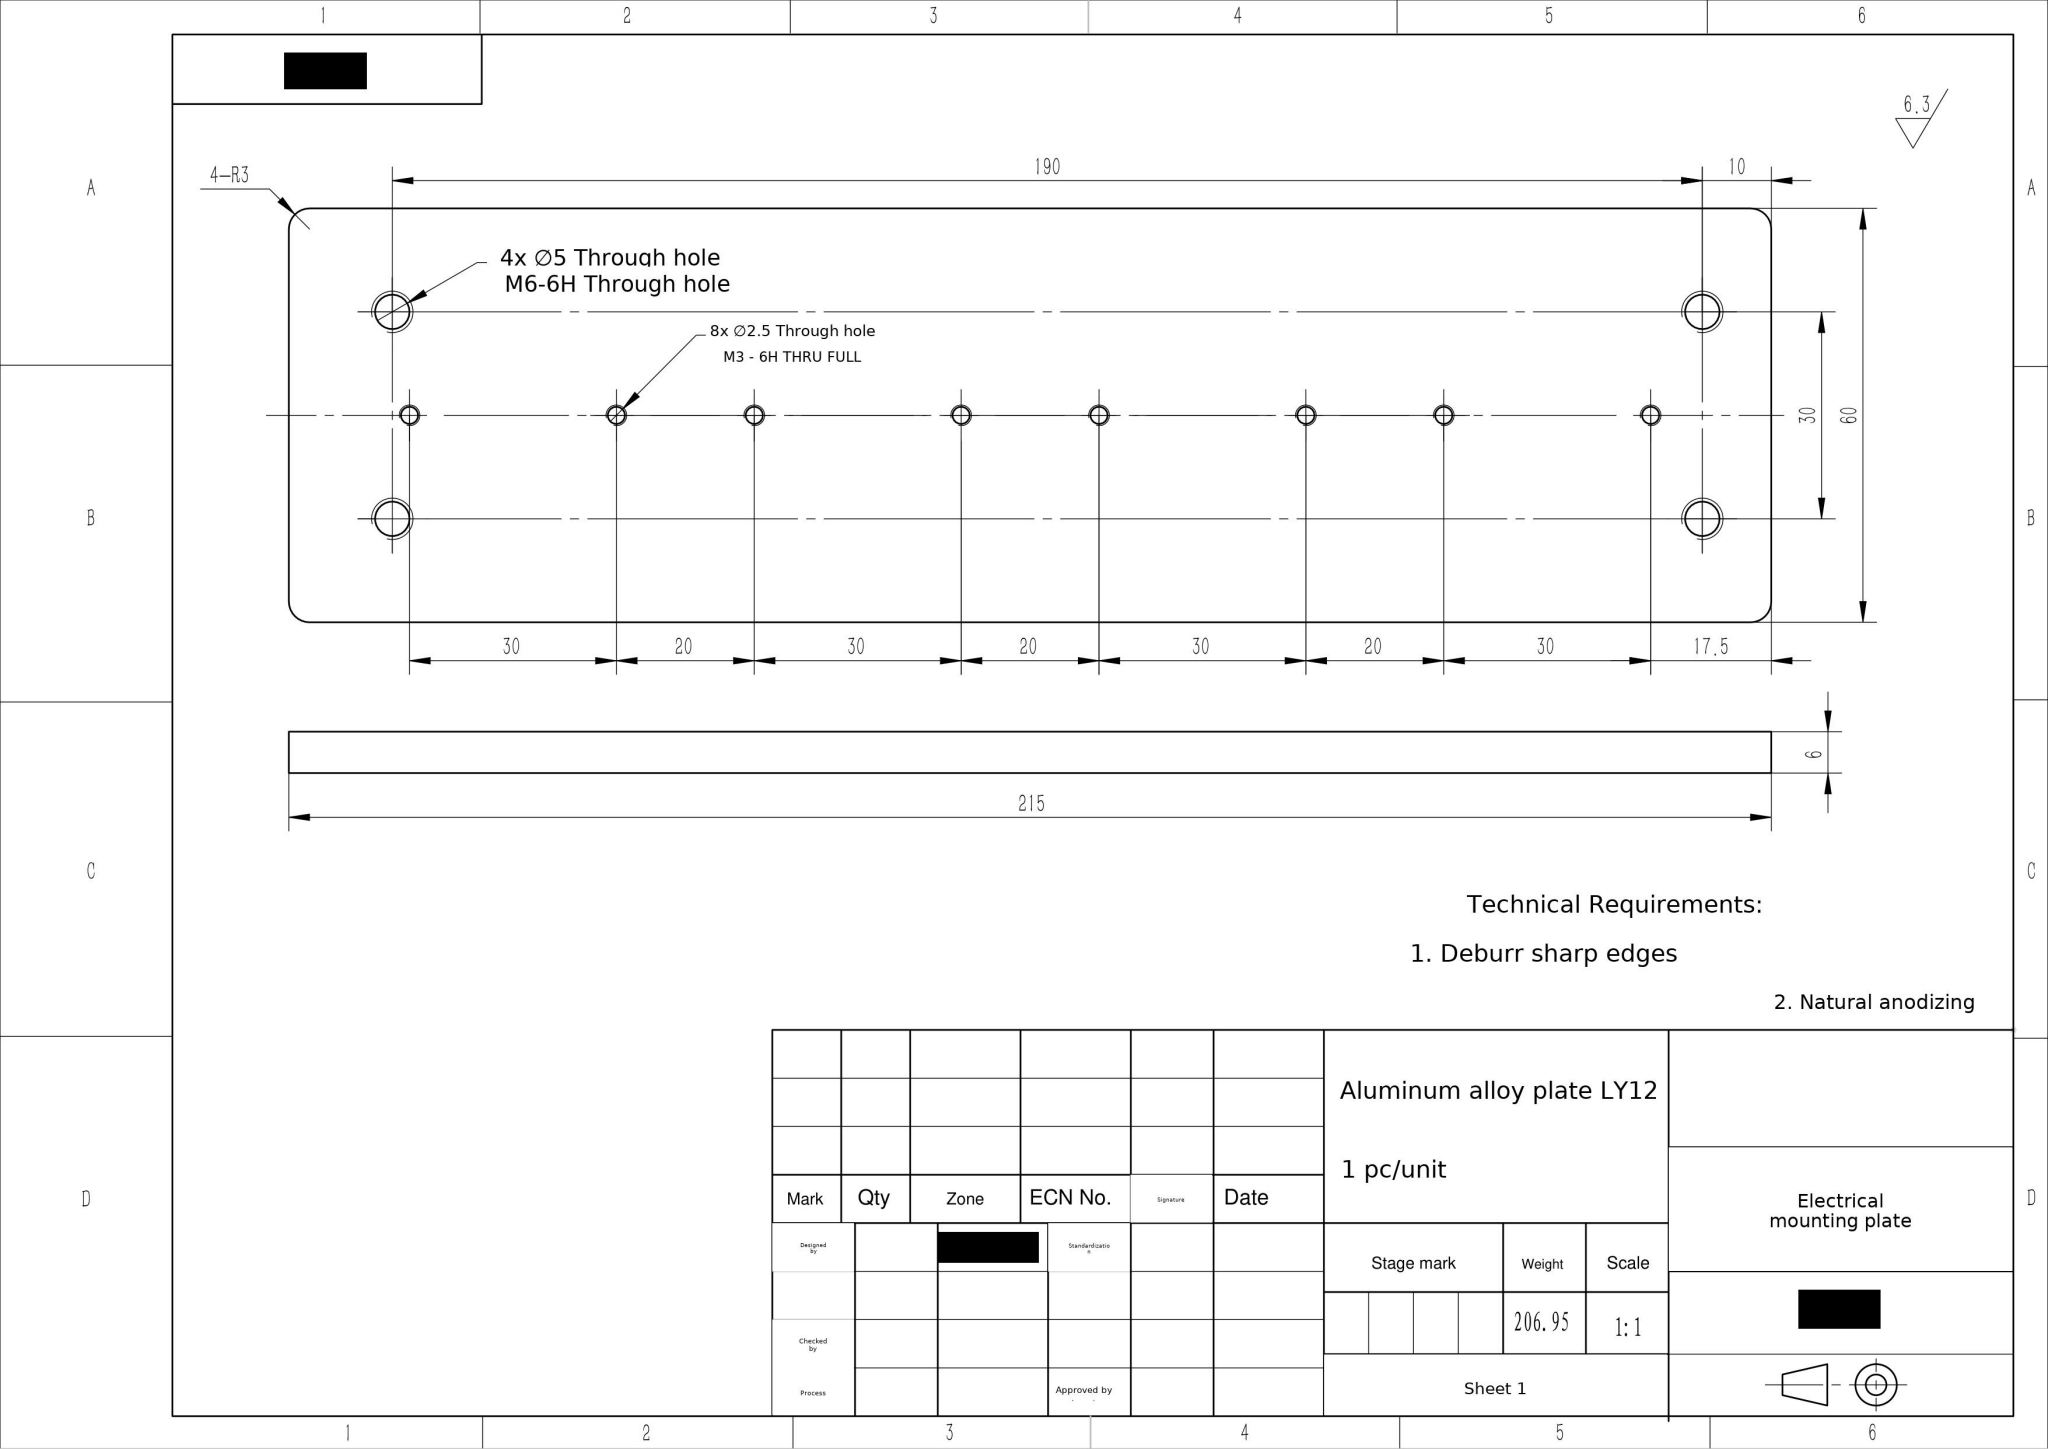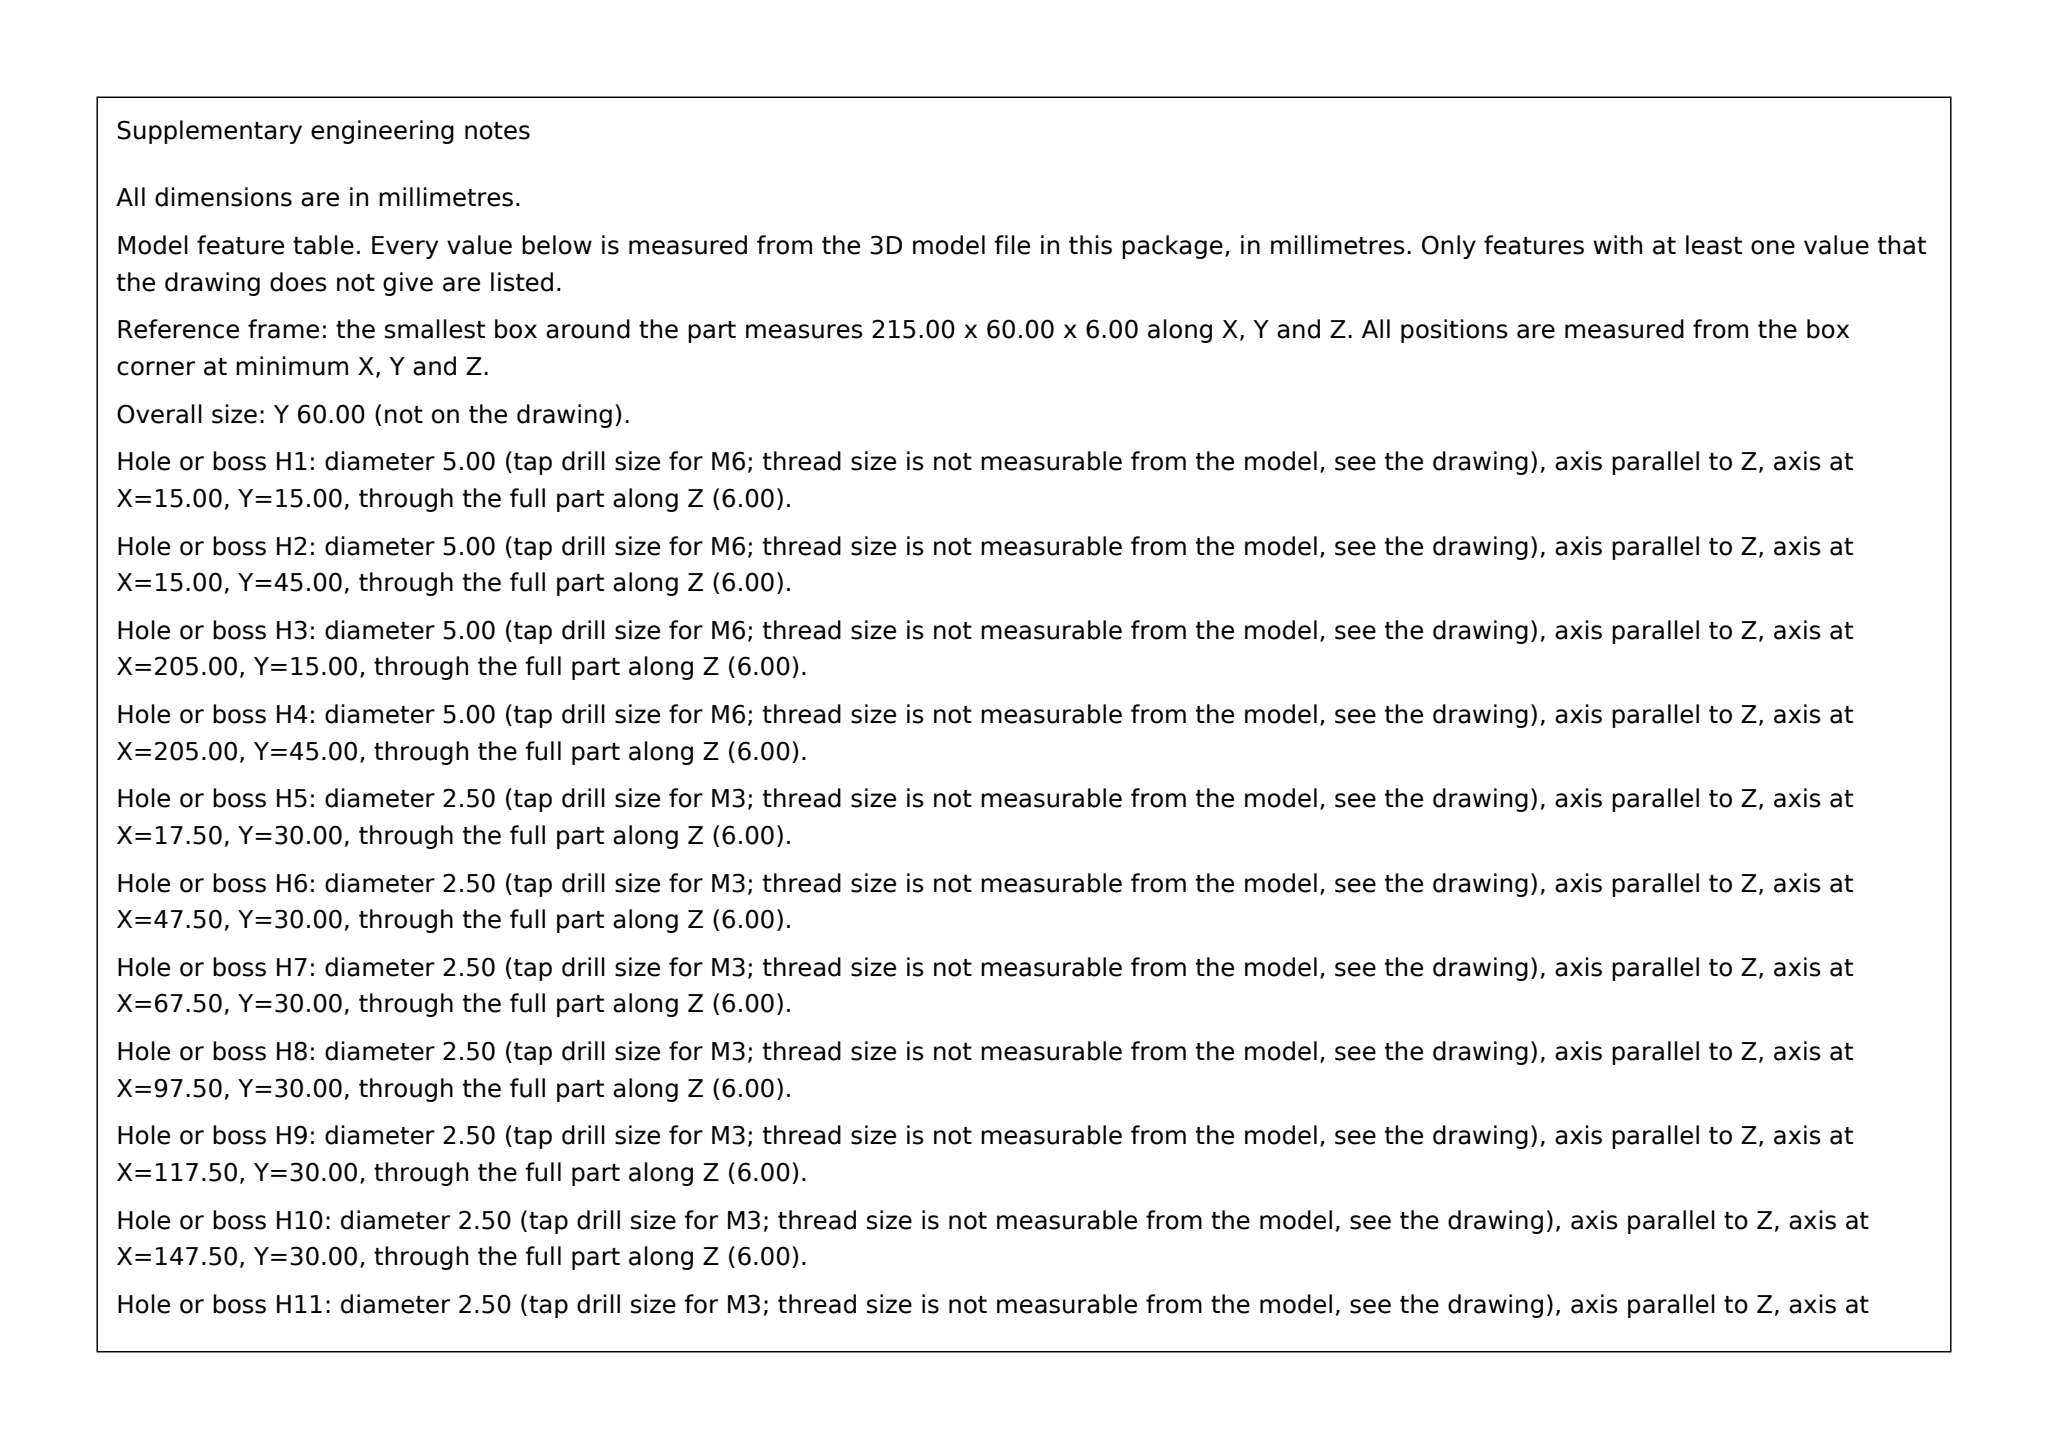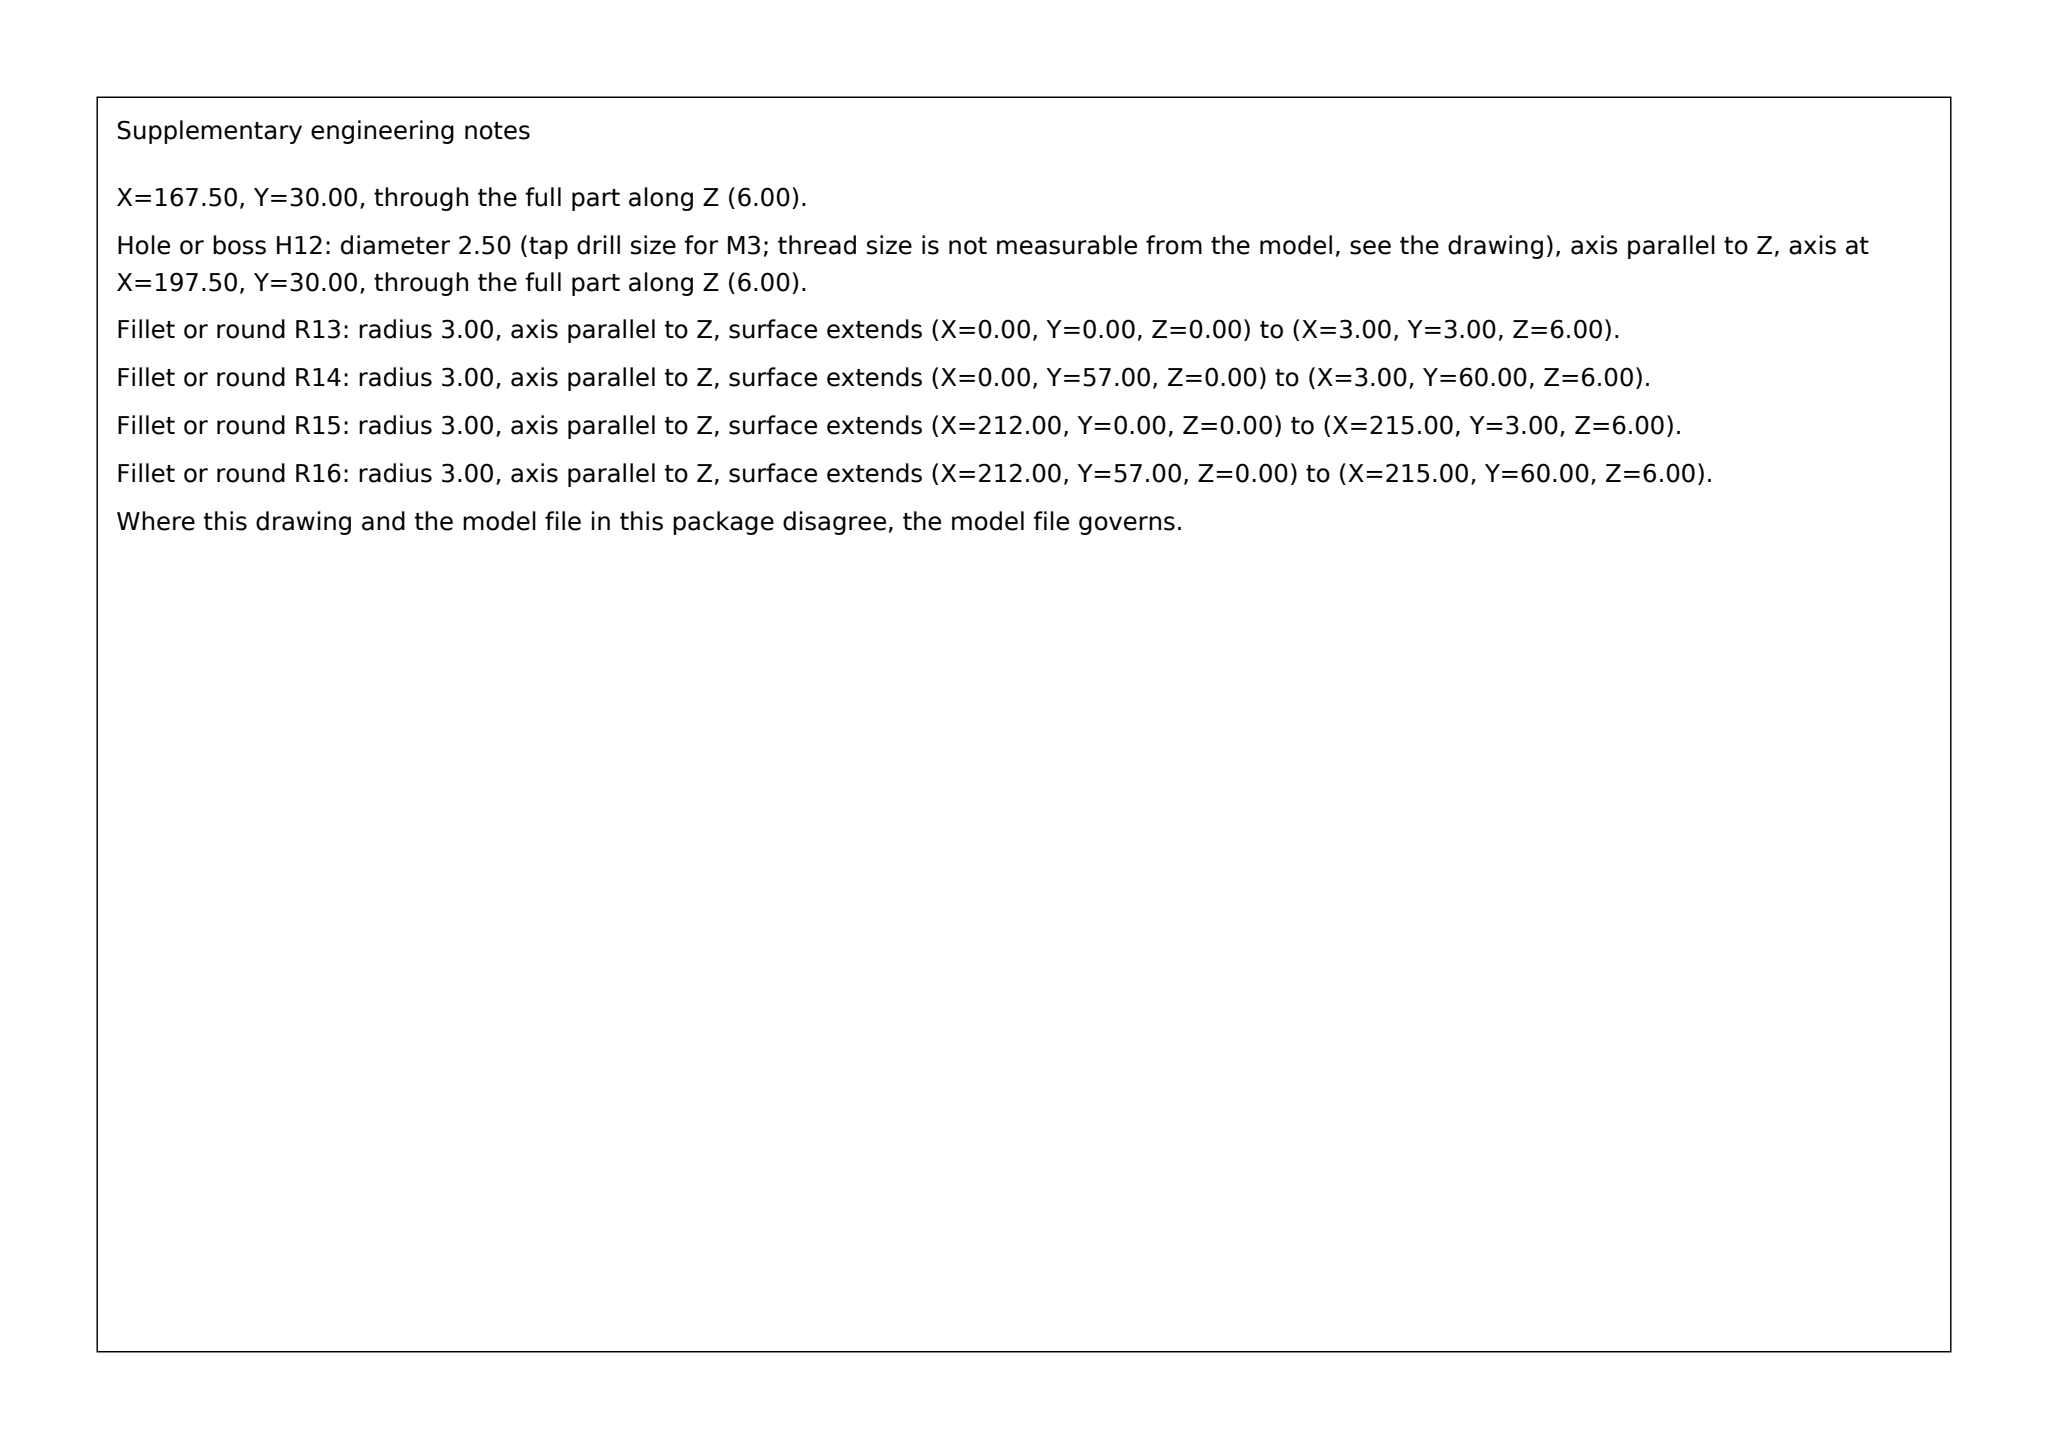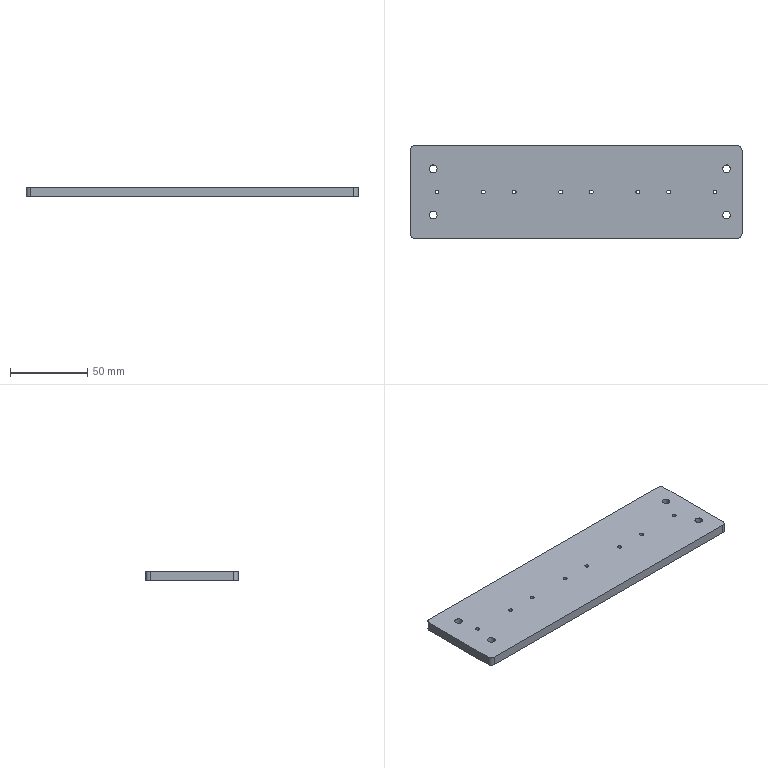Part | SolidWorks | mm | material Aluminum alloy plate LY12 | 1 solid | 34 faces | box 215 x 60 x 6 mm | volume 76647 mm3 | cylinder 28 | plane 6 | commonest cylinder face diameters 2.5 x16 5 x8 6 x4
build123d program:
from build123d import *

# Parameters (mm, degrees)
SKETCH1_W           = 215
SKETCH1_H           = 60
BOSS_EXTRUDE1_DEPTH = 6
M3_TAPPED_HOLE1_D   = 2.5
LPATTERN1_COUNT     = 4
LPATTERN1_PITCH     = 50
M6_TAPPED_HOLE2_D   = 5
FILLET1_R           = 3
LPATTERN2_COUNT     = 2
LPATTERN2_PITCH     = 30


with BuildPart() as part:
    # Sketch1 → Boss-Extrude1 (new body)
    with BuildSketch(Plane.XY):
        Rectangle(SKETCH1_W, SKETCH1_H)
    extrude(amount=BOSS_EXTRUDE1_DEPTH)

    # M3 Tapped Hole1 (through all)
    with Locations(Plane.XY.offset(6)):
        with Locations((-90, 0), (-60, 0)):
            m3_tapped_hole1 = Hole(M3_TAPPED_HOLE1_D / 2)

    # LPattern1: M3 Tapped Hole1 ×4
    with Locations(*[(i * LPATTERN1_PITCH, 0, 0) for i in range(1, LPATTERN1_COUNT)]):
        add(m3_tapped_hole1, mode=Mode.SUBTRACT)

    # M6 Tapped Hole2 (through all)
    with Locations(Plane.XY.offset(6)):
        with Locations((97.5, 15), (-92.5, 15)):
            m6_tapped_hole2 = Hole(M6_TAPPED_HOLE2_D / 2)

    # Fillet1
    fillet1_edges = [part.edges().sort_by_distance(p)[0] for p in [
        (107.5, -30, 3),
        (-107.5, -30, 3),
        (-107.5, 30, 3),
        (107.5, 30, 3),
    ]]
    fillet(fillet1_edges, radius=FILLET1_R)

    # LPattern2: M6 Tapped Hole2 ×2
    with Locations(*[(0, -i * LPATTERN2_PITCH, 0) for i in range(1, LPATTERN2_COUNT)]):
        add(m6_tapped_hole2, mode=Mode.SUBTRACT)


solid = part.part